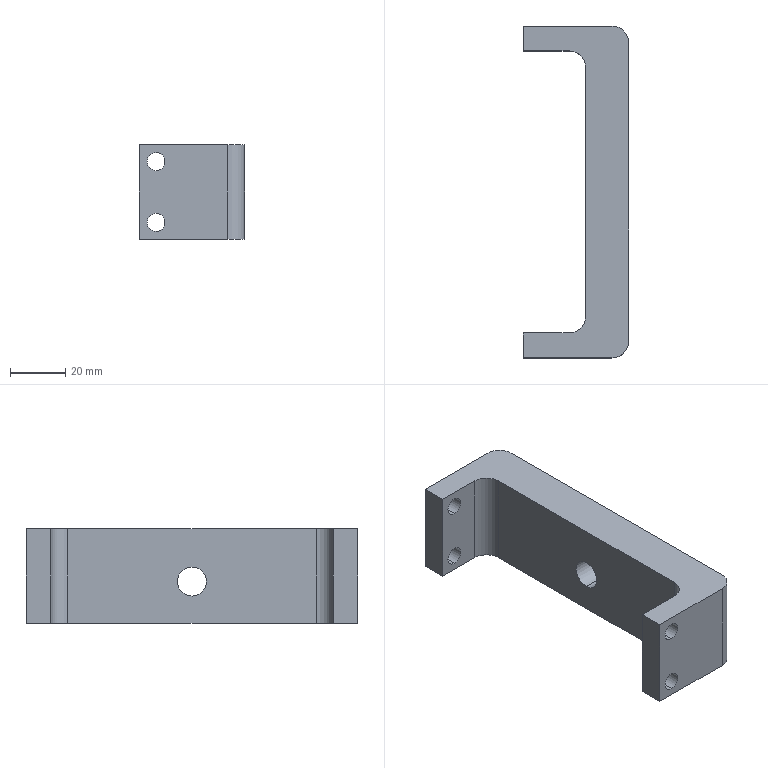CAM job | Mastercam | mm | 9 operations | part box 38 x 120 x 34
1. Facing | 20 - 63 平铣刀
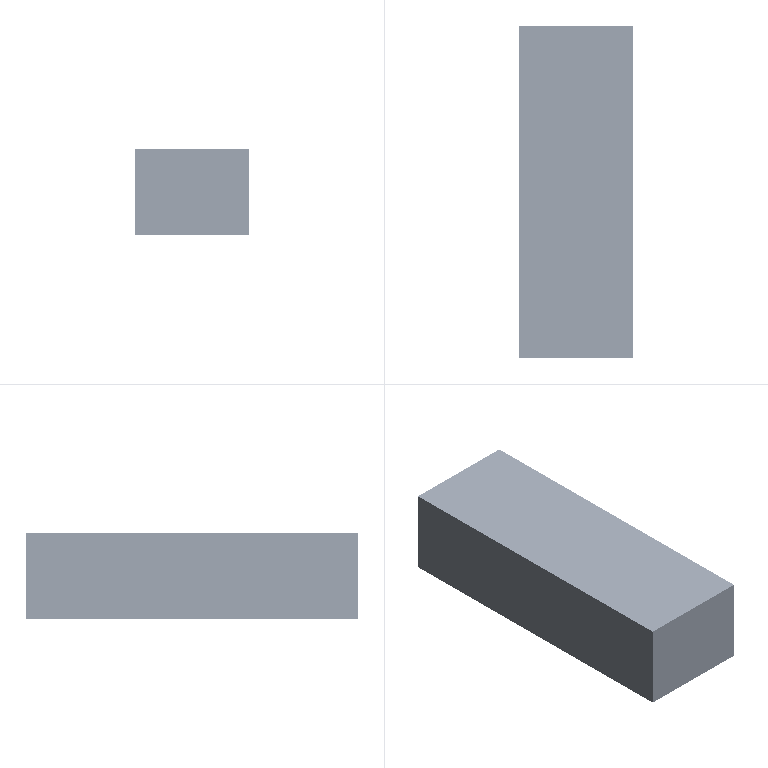2. 2D High Speed (2D Dynamic Mill) | 10 - 10 平铣刀
3. Contour (2D) | 10 - 10 平铣刀
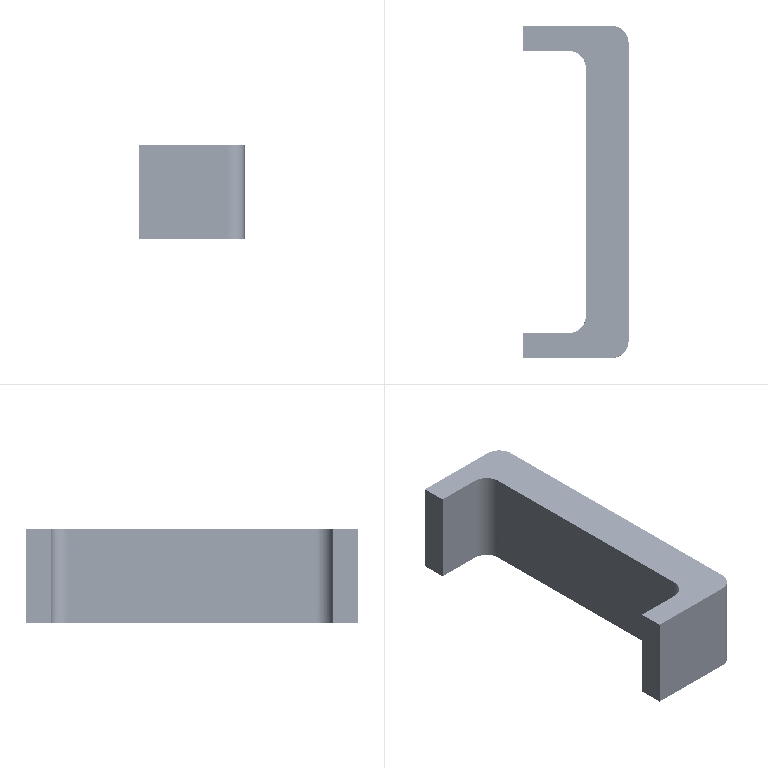4. Contour (2D chamfer) | 7 - 6 倒角刀
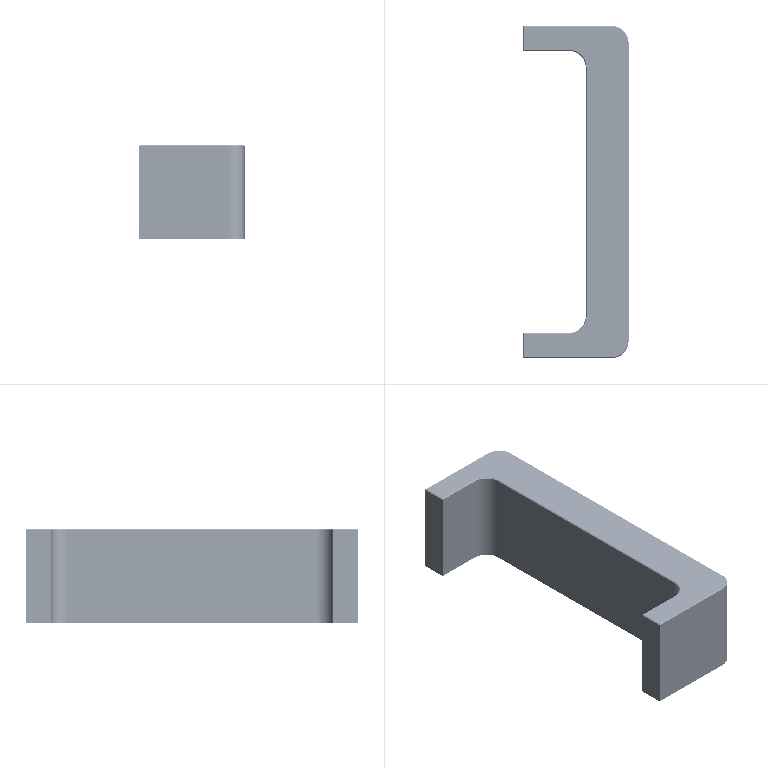5. Facing | 20 - 63 平铣刀
6. Contour (2D chamfer) | 7 - 6 倒角刀
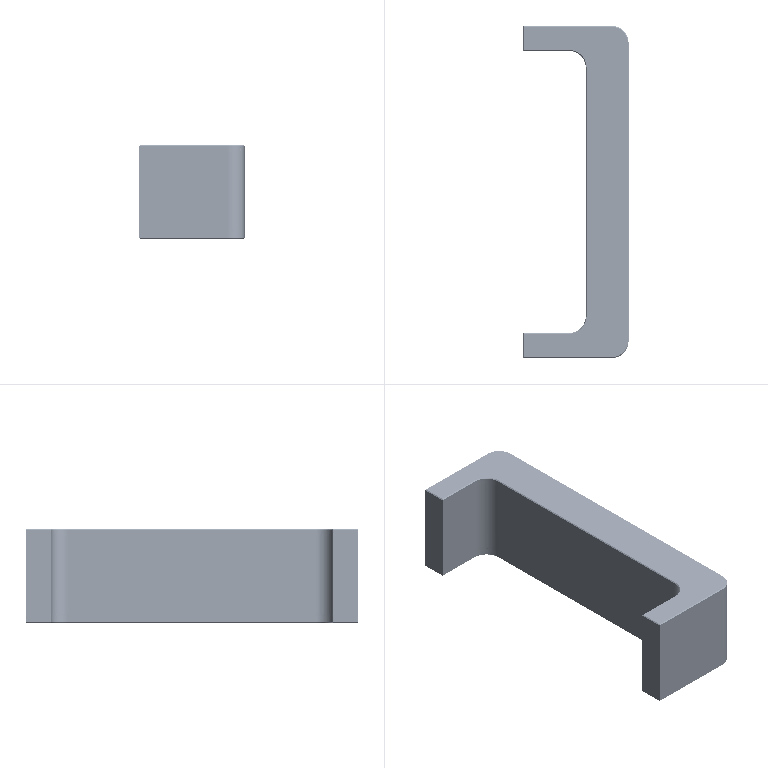7. Helix Bore | 6 - 6 平铣刀
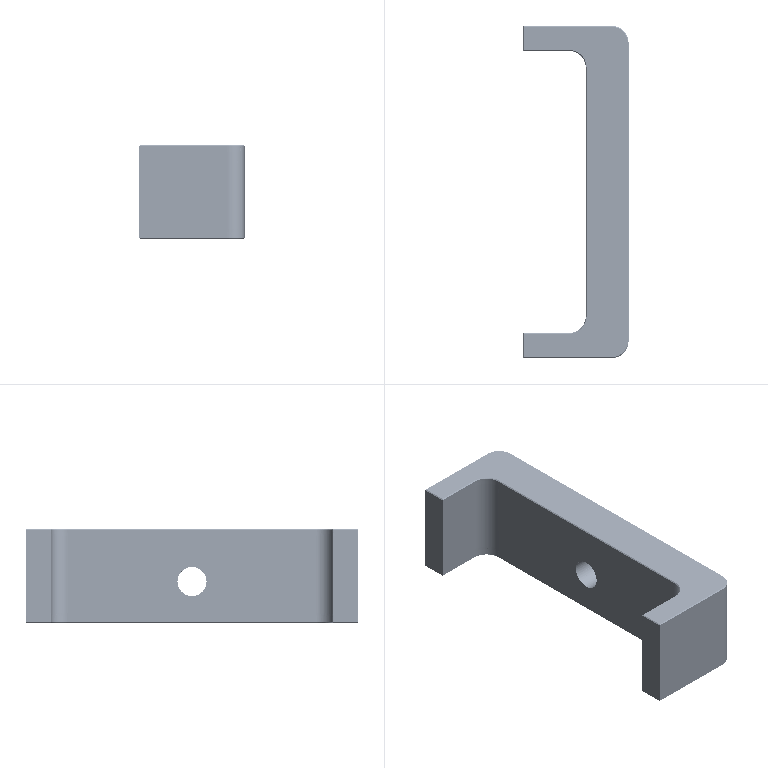8. Contour (2D chamfer) | 7 - 6 倒角刀
9. Drill/Counterbore | 7 - 6 倒角刀